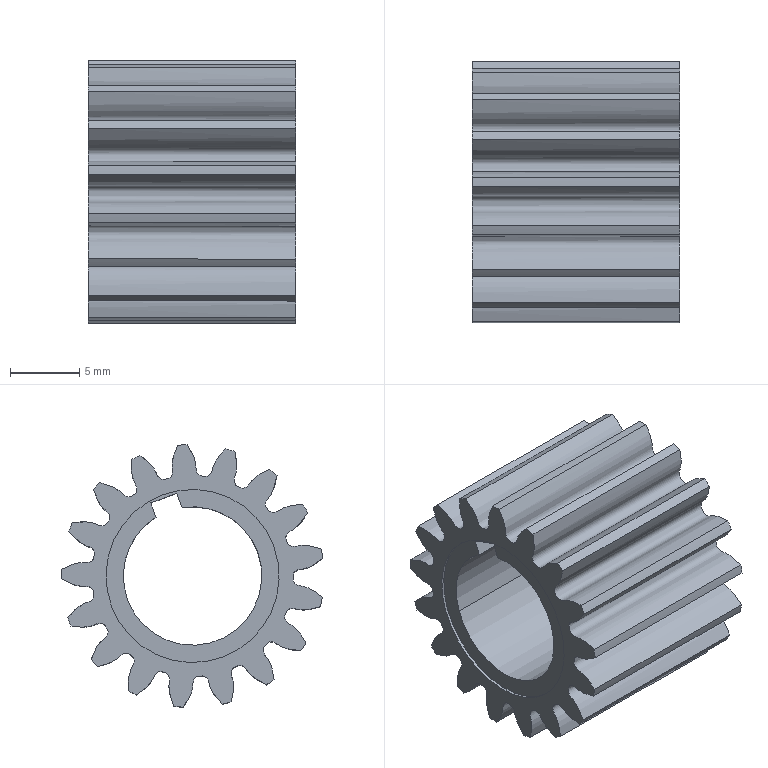Component | SolidWorks | ArmGrippingGear-1 | 1 solid | 48 faces | box 15.02 x 18.91 x 18.98 mm | volume 2167 mm3 | cylinder 24 | spline 17 | plane 7 | commonest cylinder face diameters 19 x17 12.5 x4 10 x3